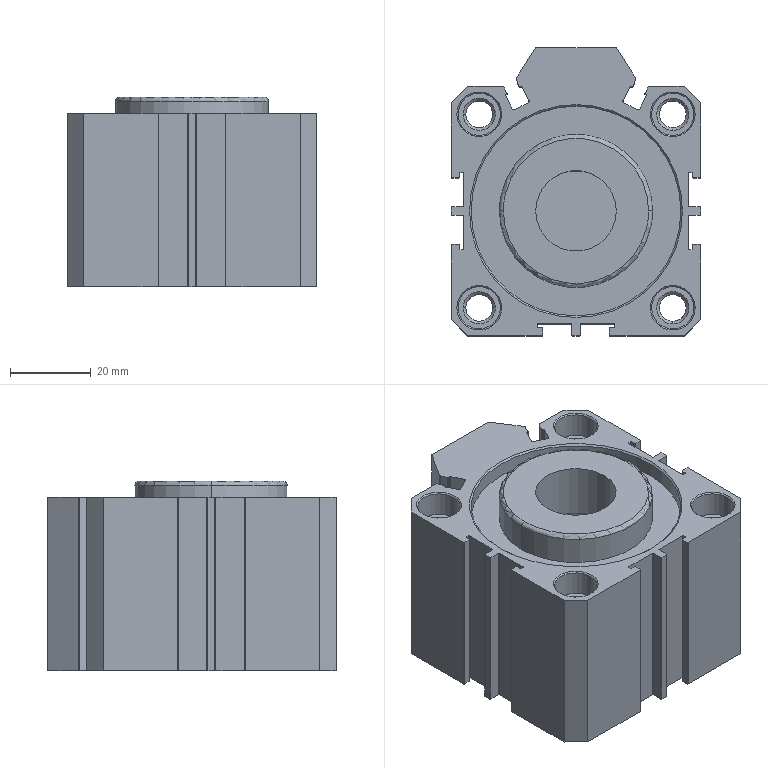Component | NX | SDAS-50X55_B_2 | 1 solid | 215 faces | volume 97197 mm3 | cylinder 94 | plane 79 | cone 40 | torus 2 | commonest cylinder face diameters 0.4 x46 10.5 x16 0.8 x10 6.647 x8 50 x4 11.445 x4 52 x2 38 x2